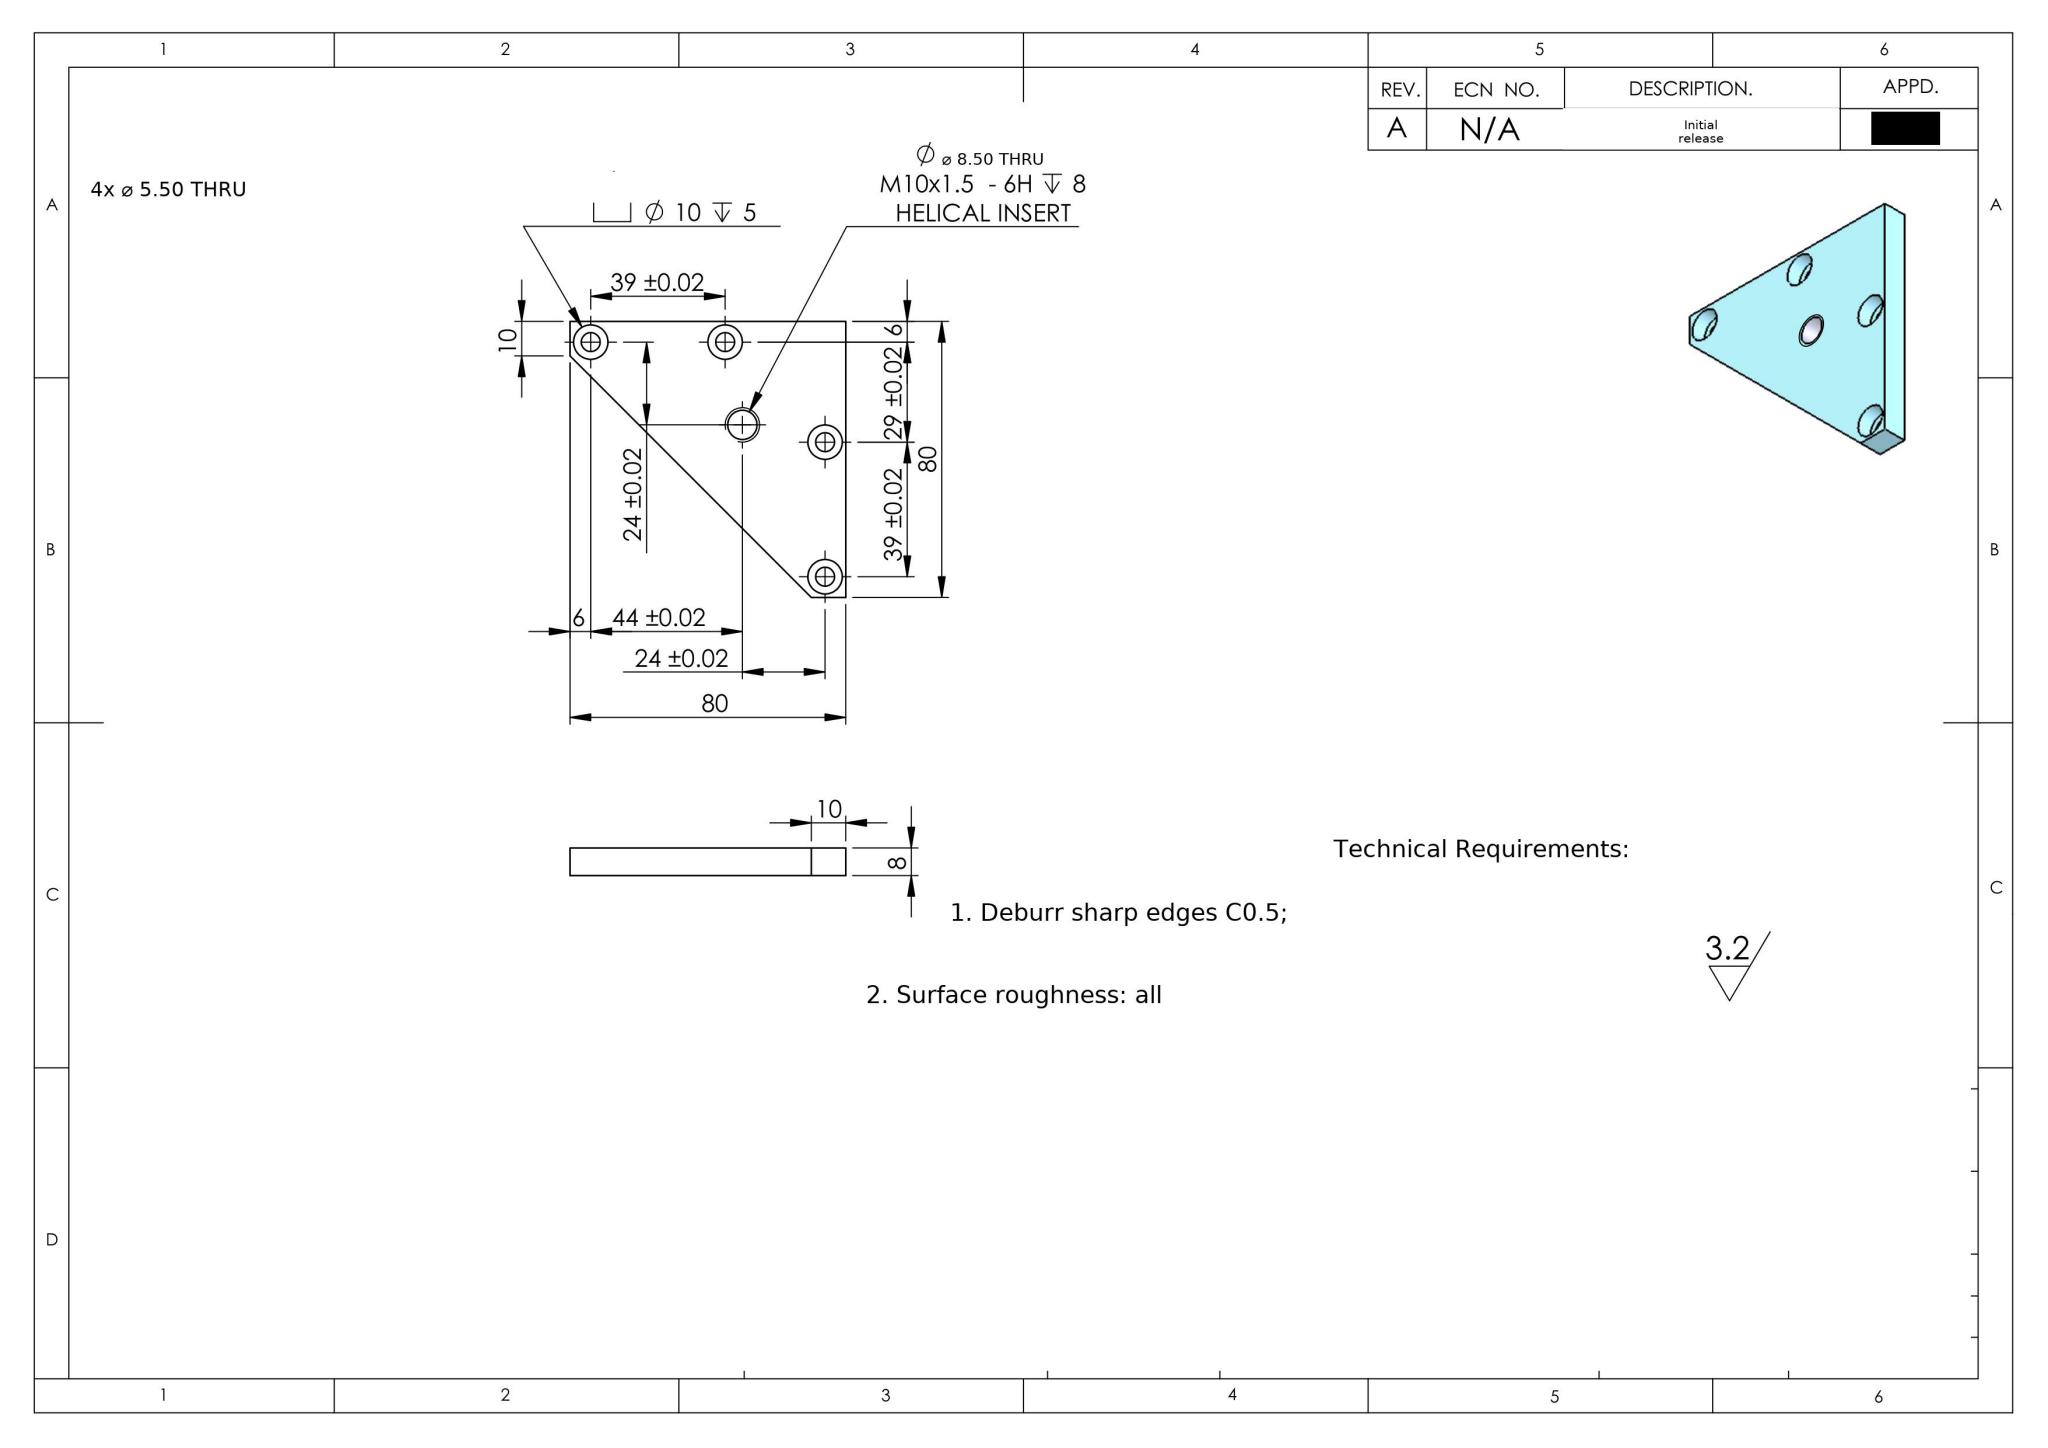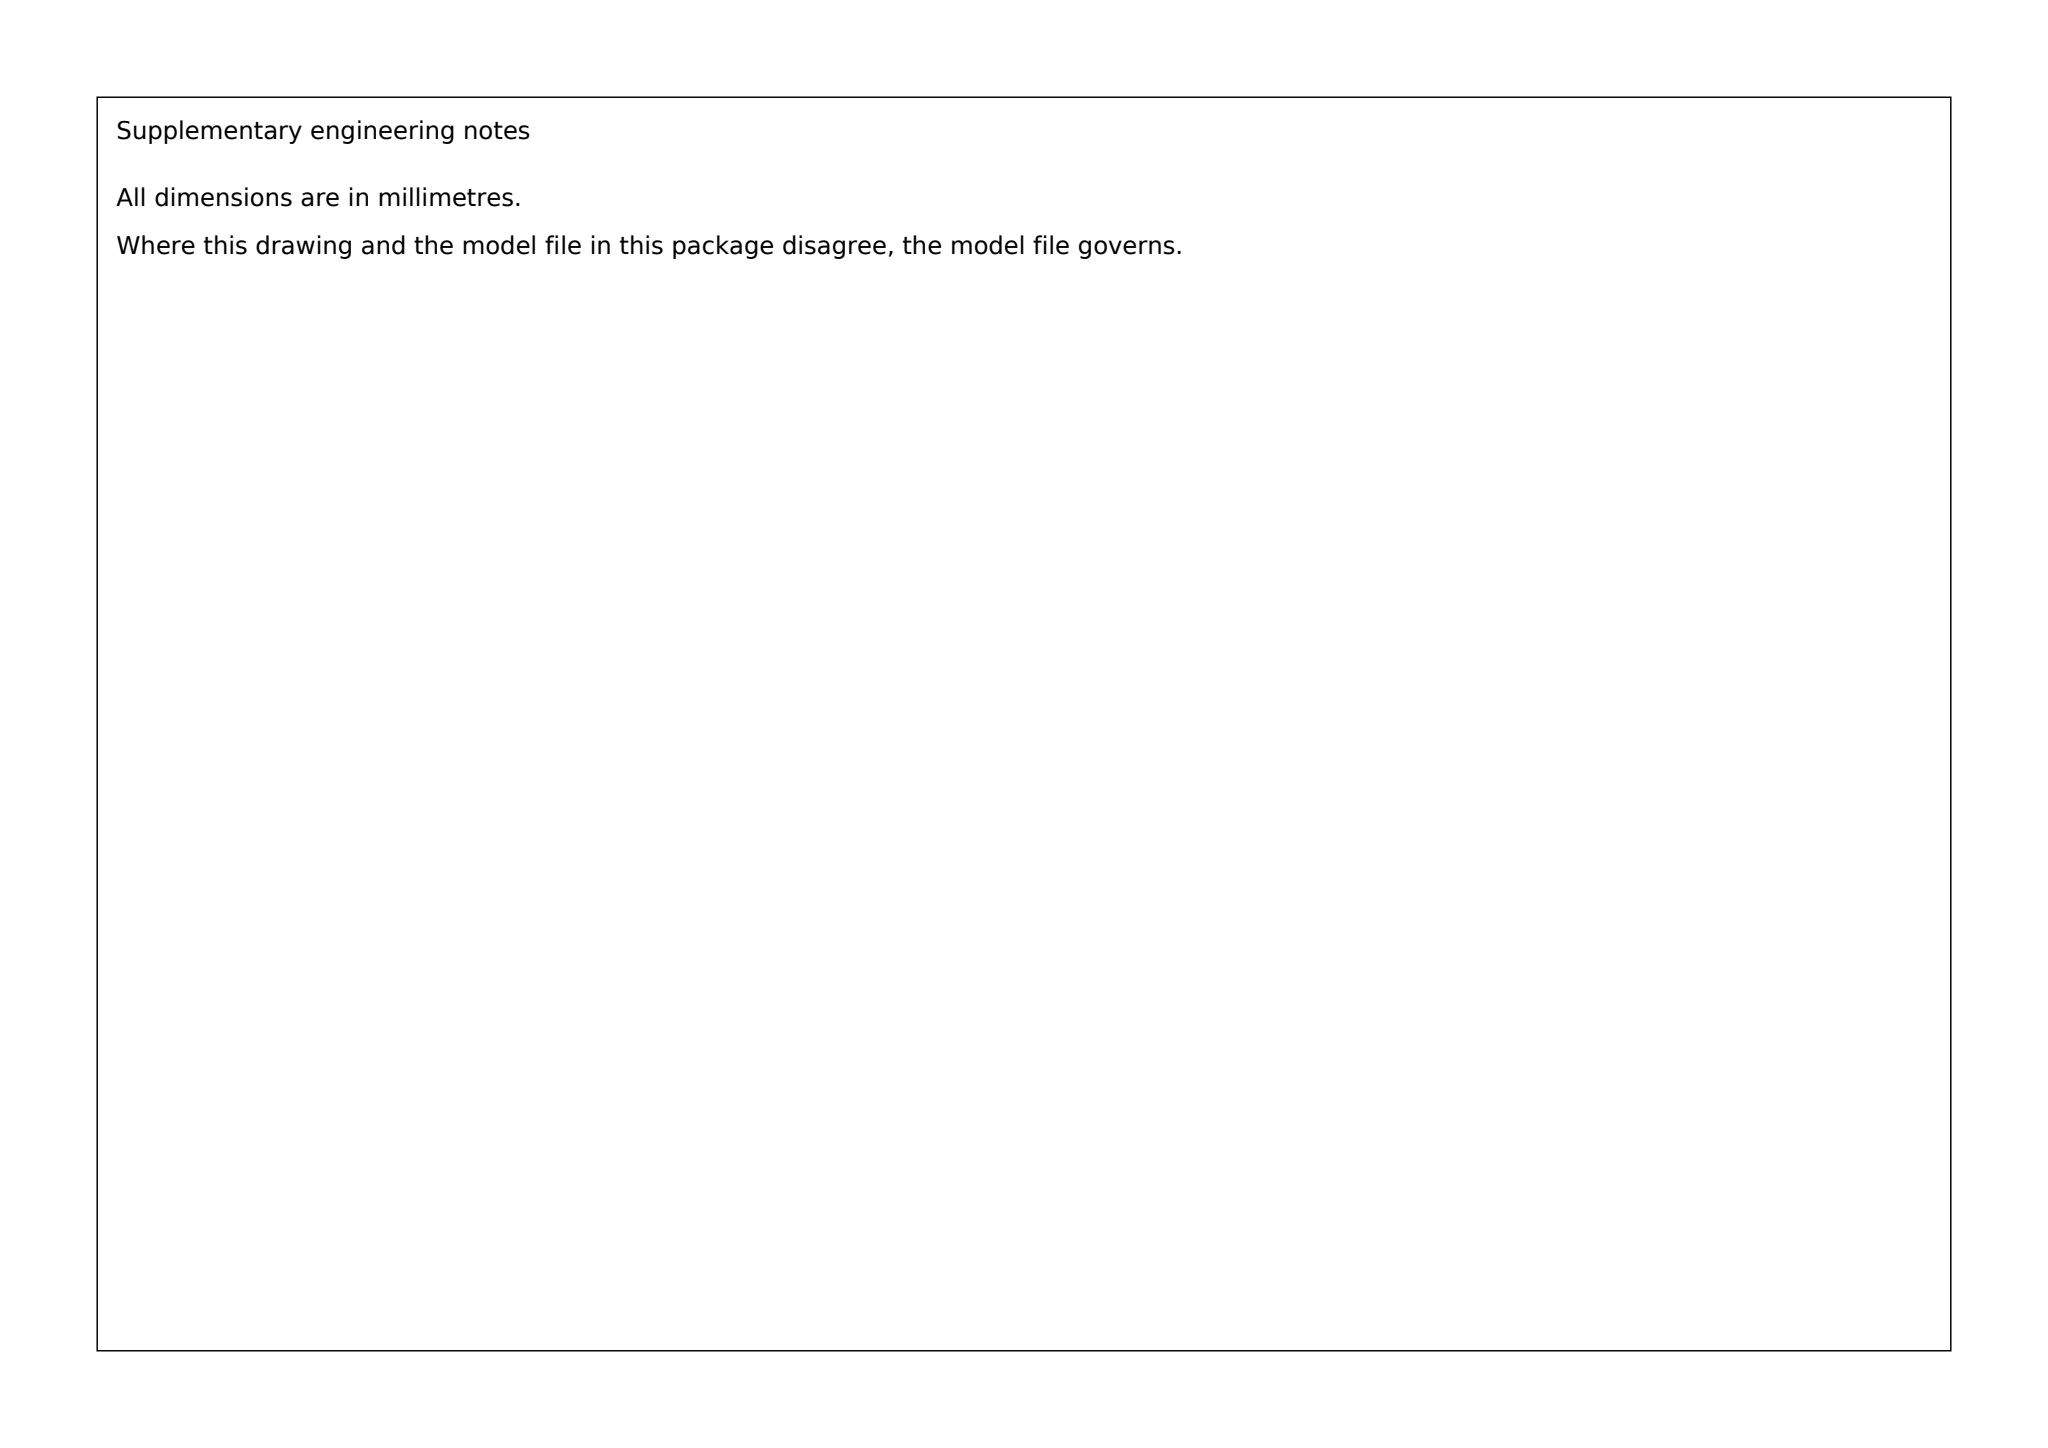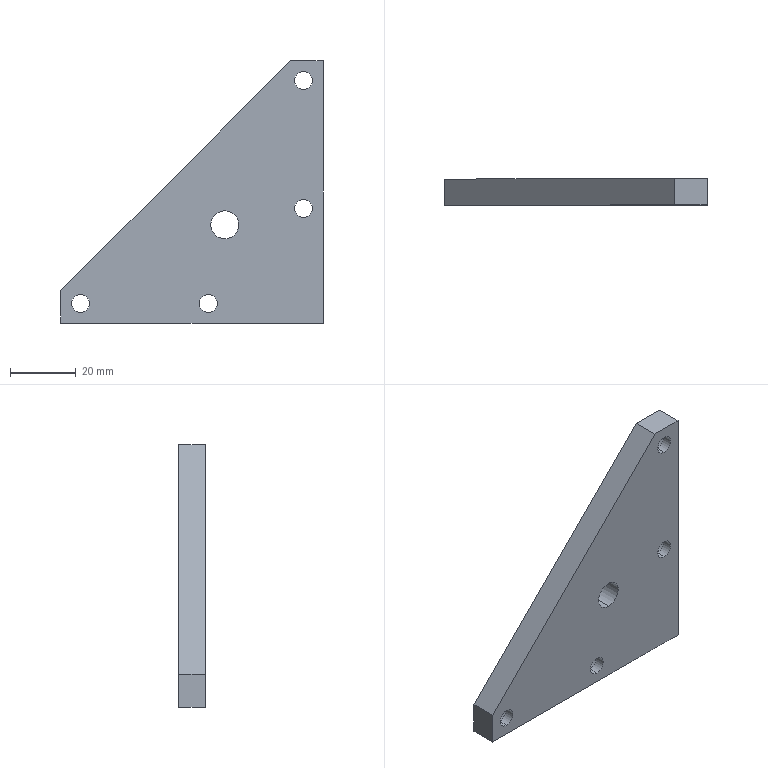Part | SolidWorks | mm | 1 solid | 29 faces | box 80 x 8 x 80 mm | volume 29290 mm3 | cylinder 18 | plane 11 | commonest cylinder face diameters 5.5 x8 10 x8 8.5 x2
build123d program:
from build123d import *

# Parameters (mm, degrees)
SKETCH1_W                                            = 80
SKETCH1_H                                            = 80
EXTRUDE1_DEPTH                                       = 8
COUNTERBORE_FOR_M5_HEX_SOCKET_HEAD_CAP_S_D           = 5.5
COUNTERBORE_FOR_M5_HEX_SOCKET_HEAD_CAP_S_CBORE_D     = 10
COUNTERBORE_FOR_M5_HEX_SOCKET_HEAD_CAP_S_CBORE_DEPTH = 5
M10_TAPPED_HOLE1_D                                   = 8.5
CUT_EXTRUDE1_REACH                                   = 115.42


with BuildPart() as part:
    # Sketch1 → Extrude1 (new body)
    with BuildSketch(Plane(origin=(0, 0, 0), x_dir=(1, 0, 0), z_dir=(0, 1, 0))):
        with Locations((40, 40)):
            Rectangle(SKETCH1_W, SKETCH1_H)
    extrude(amount=EXTRUDE1_DEPTH)

    # Counterbore for M5 Hex Socket Head Cap S (through all)
    with Locations(Plane(origin=(0, 8, 0), x_dir=(-1, 0, 0), z_dir=(0, 1, 0))):
        with Locations((-74, -45), (-74, -6), (-6, -6), (-6, -74), (-45, -74)):
            CounterBoreHole(COUNTERBORE_FOR_M5_HEX_SOCKET_HEAD_CAP_S_D / 2, COUNTERBORE_FOR_M5_HEX_SOCKET_HEAD_CAP_S_CBORE_D / 2, COUNTERBORE_FOR_M5_HEX_SOCKET_HEAD_CAP_S_CBORE_DEPTH)

    # M10 Tapped Hole1 (through all)
    with Locations(Plane(origin=(0, 8, 0), x_dir=(-1, 0, 0), z_dir=(0, 1, 0))):
        with Locations((-50, -50)):
            Hole(M10_TAPPED_HOLE1_D / 2)

    # Sketch8 → Cut-Extrude1 (cut, up to next)
    with BuildSketch(Plane(origin=(0, 8, 0), x_dir=(-1, 0, 0), z_dir=(0, 1, 0)), mode=Mode.PRIVATE) as cut_extrude1_sk1:
        Polygon((0, 0), (0, -70), (-70, 0), align=None)
    cut_extrude1_tool1 = extrude(cut_extrude1_sk1.sketch, amount=-CUT_EXTRUDE1_REACH, mode=Mode.PRIVATE) & part.part
    add(cut_extrude1_tool1.solids().sort_by_distance((23.333, 8, -23.333))[0], mode=Mode.SUBTRACT)


solid = part.part
STEP:
#1=CARTESIAN_POINT('',(50.,0.,-45.75));
#2=VERTEX_POINT('',#1);
#3=CARTESIAN_POINT('',(50.,0.,-54.25));
#4=VERTEX_POINT('',#3);
#5=CARTESIAN_POINT('',(50.,0.,-50.));
#6=DIRECTION('',(0.,-1.,0.));
#7=DIRECTION('',(0.,0.,-1.));
#8=AXIS2_PLACEMENT_3D('',#5,#6,#7);
#9=CIRCLE('',#8,4.25);
#10=EDGE_CURVE('',#2,#4,#9,.T.);
#11=ORIENTED_EDGE('',*,*,#10,.T.);
#12=CARTESIAN_POINT('',(50.,8.,-54.25));
#13=VERTEX_POINT('',#12);
#14=CARTESIAN_POINT('',(50.,8.,-54.25));
#15=DIRECTION('',(0.,1.,0.));
#16=VECTOR('',#15,1000.);
#17=LINE('',#14,#16);
#18=EDGE_CURVE('',#4,#13,#17,.T.);
#19=ORIENTED_EDGE('',*,*,#18,.T.);
#20=CARTESIAN_POINT('',(50.,8.,-45.75));
#21=VERTEX_POINT('',#20);
#22=CARTESIAN_POINT('',(50.,8.,-50.));
#23=DIRECTION('',(0.,1.,0.));
#24=DIRECTION('',(0.,0.,1.));
#25=AXIS2_PLACEMENT_3D('',#22,#23,#24);
#26=CIRCLE('',#25,4.25);
#27=EDGE_CURVE('',#13,#21,#26,.T.);
#28=ORIENTED_EDGE('',*,*,#27,.T.);
#29=CARTESIAN_POINT('',(50.,8.,-45.75));
#30=DIRECTION('',(0.,1.,0.));
#31=VECTOR('',#30,1000.);
#32=LINE('',#29,#31);
#33=EDGE_CURVE('',#2,#21,#32,.T.);
#34=ORIENTED_EDGE('',*,*,#33,.F.);
#35=EDGE_LOOP('',(#11,#19,#28,#34));
#36=FACE_OUTER_BOUND('',#35,.T.);
#37=CARTESIAN_POINT('',(50.,8.,-50.));
#38=DIRECTION('',(0.,1.,0.));
#39=DIRECTION('',(0.,0.,1.));
#40=AXIS2_PLACEMENT_3D('',#37,#38,#39);
#41=CYLINDRICAL_SURFACE('',#40,4.25);
#42=ADVANCED_FACE('',(#36),#41,.F.);
#43=CARTESIAN_POINT('',(74.,0.,-47.75));
#44=VERTEX_POINT('',#43);
#45=CARTESIAN_POINT('',(74.,0.,-42.25));
#46=VERTEX_POINT('',#45);
#47=CARTESIAN_POINT('',(74.,0.,-45.));
#48=DIRECTION('',(0.,1.,0.));
#49=DIRECTION('',(0.,0.,1.));
#50=AXIS2_PLACEMENT_3D('',#47,#48,#49);
#51=CIRCLE('',#50,2.75);
#52=EDGE_CURVE('',#44,#46,#51,.T.);
#53=ORIENTED_EDGE('',*,*,#52,.F.);
#54=CARTESIAN_POINT('',(74.,3.,-47.75));
#55=VERTEX_POINT('',#54);
#56=CARTESIAN_POINT('',(74.,8.,-47.75));
#57=DIRECTION('',(0.,1.,0.));
#58=VECTOR('',#57,1000.);
#59=LINE('',#56,#58);
#60=EDGE_CURVE('',#44,#55,#59,.T.);
#61=ORIENTED_EDGE('',*,*,#60,.T.);
#62=CARTESIAN_POINT('',(74.,3.,-42.25));
#63=VERTEX_POINT('',#62);
#64=CARTESIAN_POINT('',(74.,3.,-45.));
#65=DIRECTION('',(0.,1.,0.));
#66=DIRECTION('',(0.,0.,1.));
#67=AXIS2_PLACEMENT_3D('',#64,#65,#66);
#68=CIRCLE('',#67,2.75);
#69=EDGE_CURVE('',#55,#63,#68,.T.);
#70=ORIENTED_EDGE('',*,*,#69,.T.);
#71=CARTESIAN_POINT('',(74.,8.,-42.25));
#72=DIRECTION('',(0.,1.,0.));
#73=VECTOR('',#72,1000.);
#74=LINE('',#71,#73);
#75=EDGE_CURVE('',#46,#63,#74,.T.);
#76=ORIENTED_EDGE('',*,*,#75,.F.);
#77=EDGE_LOOP('',(#53,#61,#70,#76));
#78=FACE_OUTER_BOUND('',#77,.T.);
#79=CARTESIAN_POINT('',(74.,8.,-45.));
#80=DIRECTION('',(0.,1.,0.));
#81=DIRECTION('',(0.,0.,1.));
#82=AXIS2_PLACEMENT_3D('',#79,#80,#81);
#83=CYLINDRICAL_SURFACE('',#82,2.75);
#84=ADVANCED_FACE('',(#78),#83,.F.);
#85=CARTESIAN_POINT('',(74.,3.,-50.));
#86=VERTEX_POINT('',#85);
#87=CARTESIAN_POINT('',(74.,3.,-40.));
#88=VERTEX_POINT('',#87);
#89=CARTESIAN_POINT('',(74.,3.,-45.));
#90=DIRECTION('',(0.,1.,0.));
#91=DIRECTION('',(0.,0.,1.));
#92=AXIS2_PLACEMENT_3D('',#89,#90,#91);
#93=CIRCLE('',#92,5.);
#94=EDGE_CURVE('',#86,#88,#93,.T.);
#95=ORIENTED_EDGE('',*,*,#94,.F.);
#96=CARTESIAN_POINT('',(74.,8.,-50.));
#97=VERTEX_POINT('',#96);
#98=CARTESIAN_POINT('',(74.,8.,-50.));
#99=DIRECTION('',(0.,1.,0.));
#100=VECTOR('',#99,1000.);
#101=LINE('',#98,#100);
#102=EDGE_CURVE('',#86,#97,#101,.T.);
#103=ORIENTED_EDGE('',*,*,#102,.T.);
#104=CARTESIAN_POINT('',(74.,8.,-40.));
#105=VERTEX_POINT('',#104);
#106=CARTESIAN_POINT('',(74.,8.,-45.));
#107=DIRECTION('',(0.,1.,0.));
#108=DIRECTION('',(0.,0.,1.));
#109=AXIS2_PLACEMENT_3D('',#106,#107,#108);
#110=CIRCLE('',#109,5.);
#111=EDGE_CURVE('',#97,#105,#110,.T.);
#112=ORIENTED_EDGE('',*,*,#111,.T.);
#113=CARTESIAN_POINT('',(74.,8.,-40.));
#114=DIRECTION('',(0.,1.,0.));
#115=VECTOR('',#114,1000.);
#116=LINE('',#113,#115);
#117=EDGE_CURVE('',#88,#105,#116,.T.);
#118=ORIENTED_EDGE('',*,*,#117,.F.);
#119=EDGE_LOOP('',(#95,#103,#112,#118));
#120=FACE_OUTER_BOUND('',#119,.T.);
#121=CARTESIAN_POINT('',(74.,8.,-45.));
#122=DIRECTION('',(0.,1.,0.));
#123=DIRECTION('',(0.,0.,1.));
#124=AXIS2_PLACEMENT_3D('',#121,#122,#123);
#125=CYLINDRICAL_SURFACE('',#124,5.);
#126=ADVANCED_FACE('',(#120),#125,.F.);
#127=CARTESIAN_POINT('',(74.,0.,-8.75));
#128=VERTEX_POINT('',#127);
#129=CARTESIAN_POINT('',(74.,0.,-3.25));
#130=VERTEX_POINT('',#129);
#131=CARTESIAN_POINT('',(74.,0.,-6.));
#132=DIRECTION('',(0.,1.,0.));
#133=DIRECTION('',(0.,0.,1.));
#134=AXIS2_PLACEMENT_3D('',#131,#132,#133);
#135=CIRCLE('',#134,2.75);
#136=EDGE_CURVE('',#128,#130,#135,.T.);
#137=ORIENTED_EDGE('',*,*,#136,.F.);
#138=CARTESIAN_POINT('',(74.,3.,-8.75));
#139=VERTEX_POINT('',#138);
#140=CARTESIAN_POINT('',(74.,8.,-8.75));
#141=DIRECTION('',(0.,1.,0.));
#142=VECTOR('',#141,1000.);
#143=LINE('',#140,#142);
#144=EDGE_CURVE('',#128,#139,#143,.T.);
#145=ORIENTED_EDGE('',*,*,#144,.T.);
#146=CARTESIAN_POINT('',(74.,3.,-3.25));
#147=VERTEX_POINT('',#146);
#148=CARTESIAN_POINT('',(74.,3.,-6.));
#149=DIRECTION('',(0.,1.,0.));
#150=DIRECTION('',(0.,0.,1.));
#151=AXIS2_PLACEMENT_3D('',#148,#149,#150);
#152=CIRCLE('',#151,2.75);
#153=EDGE_CURVE('',#139,#147,#152,.T.);
#154=ORIENTED_EDGE('',*,*,#153,.T.);
#155=CARTESIAN_POINT('',(74.,8.,-3.25));
#156=DIRECTION('',(0.,1.,0.));
#157=VECTOR('',#156,1000.);
#158=LINE('',#155,#157);
#159=EDGE_CURVE('',#130,#147,#158,.T.);
#160=ORIENTED_EDGE('',*,*,#159,.F.);
#161=EDGE_LOOP('',(#137,#145,#154,#160));
#162=FACE_OUTER_BOUND('',#161,.T.);
#163=CARTESIAN_POINT('',(74.,8.,-6.));
#164=DIRECTION('',(0.,1.,0.));
#165=DIRECTION('',(0.,0.,1.));
#166=AXIS2_PLACEMENT_3D('',#163,#164,#165);
#167=CYLINDRICAL_SURFACE('',#166,2.75);
#168=ADVANCED_FACE('',(#162),#167,.F.);
#169=CARTESIAN_POINT('',(74.,3.,-11.));
#170=VERTEX_POINT('',#169);
#171=CARTESIAN_POINT('',(74.,3.,-1.));
#172=VERTEX_POINT('',#171);
#173=CARTESIAN_POINT('',(74.,3.,-6.));
#174=DIRECTION('',(0.,1.,0.));
#175=DIRECTION('',(0.,0.,1.));
#176=AXIS2_PLACEMENT_3D('',#173,#174,#175);
#177=CIRCLE('',#176,5.);
#178=EDGE_CURVE('',#170,#172,#177,.T.);
#179=ORIENTED_EDGE('',*,*,#178,.F.);
#180=CARTESIAN_POINT('',(74.,8.,-11.));
#181=VERTEX_POINT('',#180);
#182=CARTESIAN_POINT('',(74.,8.,-11.));
#183=DIRECTION('',(0.,1.,0.));
#184=VECTOR('',#183,1000.);
#185=LINE('',#182,#184);
#186=EDGE_CURVE('',#170,#181,#185,.T.);
#187=ORIENTED_EDGE('',*,*,#186,.T.);
#188=CARTESIAN_POINT('',(74.,8.,-1.));
#189=VERTEX_POINT('',#188);
#190=CARTESIAN_POINT('',(74.,8.,-6.));
#191=DIRECTION('',(0.,1.,0.));
#192=DIRECTION('',(0.,0.,1.));
#193=AXIS2_PLACEMENT_3D('',#190,#191,#192);
#194=CIRCLE('',#193,5.);
#195=EDGE_CURVE('',#181,#189,#194,.T.);
#196=ORIENTED_EDGE('',*,*,#195,.T.);
#197=CARTESIAN_POINT('',(74.,8.,-1.));
#198=DIRECTION('',(0.,1.,0.));
#199=VECTOR('',#198,1000.);
#200=LINE('',#197,#199);
#201=EDGE_CURVE('',#172,#189,#200,.T.);
#202=ORIENTED_EDGE('',*,*,#201,.F.);
#203=EDGE_LOOP('',(#179,#187,#196,#202));
#204=FACE_OUTER_BOUND('',#203,.T.);
#205=CARTESIAN_POINT('',(74.,8.,-6.));
#206=DIRECTION('',(0.,1.,0.));
#207=DIRECTION('',(0.,0.,1.));
#208=AXIS2_PLACEMENT_3D('',#205,#206,#207);
#209=CYLINDRICAL_SURFACE('',#208,5.);
#210=ADVANCED_FACE('',(#204),#209,.F.);
#211=CARTESIAN_POINT('',(6.,0.,-76.75));
#212=VERTEX_POINT('',#211);
#213=CARTESIAN_POINT('',(6.,0.,-71.25));
#214=VERTEX_POINT('',#213);
#215=CARTESIAN_POINT('',(6.,0.,-74.));
#216=DIRECTION('',(0.,1.,0.));
#217=DIRECTION('',(0.,0.,1.));
#218=AXIS2_PLACEMENT_3D('',#215,#216,#217);
#219=CIRCLE('',#218,2.75);
#220=EDGE_CURVE('',#212,#214,#219,.T.);
#221=ORIENTED_EDGE('',*,*,#220,.F.);
#222=CARTESIAN_POINT('',(6.,3.,-76.75));
#223=VERTEX_POINT('',#222);
#224=CARTESIAN_POINT('',(6.,8.,-76.75));
#225=DIRECTION('',(0.,1.,0.));
#226=VECTOR('',#225,1000.);
#227=LINE('',#224,#226);
#228=EDGE_CURVE('',#212,#223,#227,.T.);
#229=ORIENTED_EDGE('',*,*,#228,.T.);
#230=CARTESIAN_POINT('',(6.,3.,-71.25));
#231=VERTEX_POINT('',#230);
#232=CARTESIAN_POINT('',(6.,3.,-74.));
#233=DIRECTION('',(0.,1.,0.));
#234=DIRECTION('',(0.,0.,1.));
#235=AXIS2_PLACEMENT_3D('',#232,#233,#234);
#236=CIRCLE('',#235,2.75);
#237=EDGE_CURVE('',#223,#231,#236,.T.);
#238=ORIENTED_EDGE('',*,*,#237,.T.);
#239=CARTESIAN_POINT('',(6.,8.,-71.25));
#240=DIRECTION('',(0.,1.,0.));
#241=VECTOR('',#240,1000.);
#242=LINE('',#239,#241);
#243=EDGE_CURVE('',#214,#231,#242,.T.);
#244=ORIENTED_EDGE('',*,*,#243,.F.);
#245=EDGE_LOOP('',(#221,#229,#238,#244));
#246=FACE_OUTER_BOUND('',#245,.T.);
#247=CARTESIAN_POINT('',(6.,8.,-74.));
#248=DIRECTION('',(0.,1.,0.));
#249=DIRECTION('',(0.,0.,1.));
#250=AXIS2_PLACEMENT_3D('',#247,#248,#249);
#251=CYLINDRICAL_SURFACE('',#250,2.75);
#252=ADVANCED_FACE('',(#246),#251,.F.);
#253=CARTESIAN_POINT('',(6.,3.,-79.));
#254=VERTEX_POINT('',#253);
#255=CARTESIAN_POINT('',(6.,3.,-69.));
#256=VERTEX_POINT('',#255);
#257=CARTESIAN_POINT('',(6.,3.,-74.));
#258=DIRECTION('',(0.,1.,0.));
#259=DIRECTION('',(0.,0.,1.));
#260=AXIS2_PLACEMENT_3D('',#257,#258,#259);
#261=CIRCLE('',#260,5.);
#262=EDGE_CURVE('',#254,#256,#261,.T.);
#263=ORIENTED_EDGE('',*,*,#262,.F.);
#264=CARTESIAN_POINT('',(6.,8.,-79.));
#265=VERTEX_POINT('',#264);
#266=CARTESIAN_POINT('',(6.,8.,-79.));
#267=DIRECTION('',(0.,1.,0.));
#268=VECTOR('',#267,1000.);
#269=LINE('',#266,#268);
#270=EDGE_CURVE('',#254,#265,#269,.T.);
#271=ORIENTED_EDGE('',*,*,#270,.T.);
#272=CARTESIAN_POINT('',(6.,8.,-69.));
#273=VERTEX_POINT('',#272);
#274=CARTESIAN_POINT('',(6.,8.,-74.));
#275=DIRECTION('',(0.,1.,0.));
#276=DIRECTION('',(0.,0.,1.));
#277=AXIS2_PLACEMENT_3D('',#274,#275,#276);
#278=CIRCLE('',#277,5.);
#279=EDGE_CURVE('',#265,#273,#278,.T.);
#280=ORIENTED_EDGE('',*,*,#279,.T.);
#281=CARTESIAN_POINT('',(6.,8.,-69.));
#282=DIRECTION('',(0.,1.,0.));
#283=VECTOR('',#282,1000.);
#284=LINE('',#281,#283);
#285=EDGE_CURVE('',#256,#273,#284,.T.);
#286=ORIENTED_EDGE('',*,*,#285,.F.);
#287=EDGE_LOOP('',(#263,#271,#280,#286));
#288=FACE_OUTER_BOUND('',#287,.T.);
#289=CARTESIAN_POINT('',(6.,8.,-74.));
#290=DIRECTION('',(0.,1.,0.));
#291=DIRECTION('',(0.,0.,1.));
#292=AXIS2_PLACEMENT_3D('',#289,#290,#291);
#293=CYLINDRICAL_SURFACE('',#292,5.);
#294=ADVANCED_FACE('',(#288),#293,.F.);
#295=CARTESIAN_POINT('',(45.,0.,-76.75));
#296=VERTEX_POINT('',#295);
#297=CARTESIAN_POINT('',(45.,0.,-71.25));
#298=VERTEX_POINT('',#297);
#299=CARTESIAN_POINT('',(45.,0.,-74.));
#300=DIRECTION('',(0.,1.,0.));
#301=DIRECTION('',(0.,0.,1.));
#302=AXIS2_PLACEMENT_3D('',#299,#300,#301);
#303=CIRCLE('',#302,2.75);
#304=EDGE_CURVE('',#296,#298,#303,.T.);
#305=ORIENTED_EDGE('',*,*,#304,.F.);
#306=CARTESIAN_POINT('',(45.,3.,-76.75));
#307=VERTEX_POINT('',#306);
#308=CARTESIAN_POINT('',(45.,8.,-76.75));
#309=DIRECTION('',(0.,1.,0.));
#310=VECTOR('',#309,1000.);
#311=LINE('',#308,#310);
#312=EDGE_CURVE('',#296,#307,#311,.T.);
#313=ORIENTED_EDGE('',*,*,#312,.T.);
#314=CARTESIAN_POINT('',(45.,3.,-71.25));
#315=VERTEX_POINT('',#314);
#316=CARTESIAN_POINT('',(45.,3.,-74.));
#317=DIRECTION('',(0.,1.,0.));
#318=DIRECTION('',(0.,0.,1.));
#319=AXIS2_PLACEMENT_3D('',#316,#317,#318);
#320=CIRCLE('',#319,2.75);
#321=EDGE_CURVE('',#307,#315,#320,.T.);
#322=ORIENTED_EDGE('',*,*,#321,.T.);
#323=CARTESIAN_POINT('',(45.,8.,-71.25));
#324=DIRECTION('',(0.,1.,0.));
#325=VECTOR('',#324,1000.);
#326=LINE('',#323,#325);
#327=EDGE_CURVE('',#298,#315,#326,.T.);
#328=ORIENTED_EDGE('',*,*,#327,.F.);
#329=EDGE_LOOP('',(#305,#313,#322,#328));
#330=FACE_OUTER_BOUND('',#329,.T.);
#331=CARTESIAN_POINT('',(45.,8.,-74.));
#332=DIRECTION('',(0.,1.,0.));
#333=DIRECTION('',(0.,0.,1.));
#334=AXIS2_PLACEMENT_3D('',#331,#332,#333);
#335=CYLINDRICAL_SURFACE('',#334,2.75);
#336=ADVANCED_FACE('',(#330),#335,.F.);
#337=CARTESIAN_POINT('',(45.,3.,-79.));
#338=VERTEX_POINT('',#337);
#339=CARTESIAN_POINT('',(45.,3.,-69.));
#340=VERTEX_POINT('',#339);
#341=CARTESIAN_POINT('',(45.,3.,-74.));
#342=DIRECTION('',(0.,1.,0.));
#343=DIRECTION('',(0.,0.,1.));
#344=AXIS2_PLACEMENT_3D('',#341,#342,#343);
#345=CIRCLE('',#344,5.);
#346=EDGE_CURVE('',#338,#340,#345,.T.);
#347=ORIENTED_EDGE('',*,*,#346,.F.);
#348=CARTESIAN_POINT('',(45.,8.,-79.));
#349=VERTEX_POINT('',#348);
#350=CARTESIAN_POINT('',(45.,8.,-79.));
#351=DIRECTION('',(0.,1.,0.));
#352=VECTOR('',#351,1000.);
#353=LINE('',#350,#352);
#354=EDGE_CURVE('',#338,#349,#353,.T.);
#355=ORIENTED_EDGE('',*,*,#354,.T.);
#356=CARTESIAN_POINT('',(45.,8.,-69.));
#357=VERTEX_POINT('',#356);
#358=CARTESIAN_POINT('',(45.,8.,-74.));
#359=DIRECTION('',(0.,1.,0.));
#360=DIRECTION('',(0.,0.,1.));
#361=AXIS2_PLACEMENT_3D('',#358,#359,#360);
#362=CIRCLE('',#361,5.);
#363=EDGE_CURVE('',#349,#357,#362,.T.);
#364=ORIENTED_EDGE('',*,*,#363,.T.);
#365=CARTESIAN_POINT('',(45.,8.,-69.));
#366=DIRECTION('',(0.,1.,0.));
#367=VECTOR('',#366,1000.);
#368=LINE('',#365,#367);
#369=EDGE_CURVE('',#340,#357,#368,.T.);
#370=ORIENTED_EDGE('',*,*,#369,.F.);
#371=EDGE_LOOP('',(#347,#355,#364,#370));
#372=FACE_OUTER_BOUND('',#371,.T.);
#373=CARTESIAN_POINT('',(45.,8.,-74.));
#374=DIRECTION('',(0.,1.,0.));
#375=DIRECTION('',(0.,0.,1.));
#376=AXIS2_PLACEMENT_3D('',#373,#374,#375);
#377=CYLINDRICAL_SURFACE('',#376,5.);
#378=ADVANCED_FACE('',(#372),#377,.F.);
#379=CARTESIAN_POINT('',(0.,8.,-80.));
#380=VERTEX_POINT('',#379);
#381=CARTESIAN_POINT('',(0.,8.,-70.));
#382=VERTEX_POINT('',#381);
#383=CARTESIAN_POINT('',(0.,8.,0.));
#384=DIRECTION('',(0.,0.,1.));
#385=VECTOR('',#384,1000.);
#386=LINE('',#383,#385);
#387=EDGE_CURVE('',#380,#382,#386,.T.);
#388=ORIENTED_EDGE('',*,*,#387,.T.);
#389=CARTESIAN_POINT('',(70.,8.,0.));
#390=VERTEX_POINT('',#389);
#391=CARTESIAN_POINT('',(0.,8.,-70.));
#392=DIRECTION('',(-0.7071,0.,-0.7071));
#393=VECTOR('',#392,1000.);
#394=LINE('',#391,#393);
#395=EDGE_CURVE('',#390,#382,#394,.T.);
#396=ORIENTED_EDGE('',*,*,#395,.F.);
#397=CARTESIAN_POINT('',(80.,8.,0.));
#398=VERTEX_POINT('',#397);
#399=CARTESIAN_POINT('',(0.,8.,0.));
#400=DIRECTION('',(1.,0.,0.));
#401=VECTOR('',#400,1000.);
#402=LINE('',#399,#401);
#403=EDGE_CURVE('',#390,#398,#402,.T.);
#404=ORIENTED_EDGE('',*,*,#403,.T.);
#405=CARTESIAN_POINT('',(80.,8.,-80.));
#406=VERTEX_POINT('',#405);
#407=CARTESIAN_POINT('',(80.,8.,0.));
#408=DIRECTION('',(0.,0.,-1.));
#409=VECTOR('',#408,1000.);
#410=LINE('',#407,#409);
#411=EDGE_CURVE('',#398,#406,#410,.T.);
#412=ORIENTED_EDGE('',*,*,#411,.T.);
#413=CARTESIAN_POINT('',(0.,8.,-80.));
#414=DIRECTION('',(-1.,0.,0.));
#415=VECTOR('',#414,1000.);
#416=LINE('',#413,#415);
#417=EDGE_CURVE('',#406,#380,#416,.T.);
#418=ORIENTED_EDGE('',*,*,#417,.T.);
#419=EDGE_LOOP('',(#388,#396,#404,#412,#418));
#420=FACE_OUTER_BOUND('',#419,.T.);
#421=CARTESIAN_POINT('',(45.,8.,-74.));
#422=DIRECTION('',(0.,1.,0.));
#423=DIRECTION('',(0.,0.,1.));
#424=AXIS2_PLACEMENT_3D('',#421,#422,#423);
#425=CIRCLE('',#424,5.);
#426=EDGE_CURVE('',#357,#349,#425,.T.);
#427=ORIENTED_EDGE('',*,*,#426,.F.);
#428=ORIENTED_EDGE('',*,*,#363,.F.);
#429=EDGE_LOOP('',(#427,#428));
#430=FACE_BOUND('',#429,.T.);
#431=CARTESIAN_POINT('',(6.,8.,-74.));
#432=DIRECTION('',(0.,1.,0.));
#433=DIRECTION('',(0.,0.,1.));
#434=AXIS2_PLACEMENT_3D('',#431,#432,#433);
#435=CIRCLE('',#434,5.);
#436=EDGE_CURVE('',#273,#265,#435,.T.);
#437=ORIENTED_EDGE('',*,*,#436,.F.);
#438=ORIENTED_EDGE('',*,*,#279,.F.);
#439=EDGE_LOOP('',(#437,#438));
#440=FACE_BOUND('',#439,.T.);
#441=CARTESIAN_POINT('',(74.,8.,-6.));
#442=DIRECTION('',(0.,1.,0.));
#443=DIRECTION('',(0.,0.,1.));
#444=AXIS2_PLACEMENT_3D('',#441,#442,#443);
#445=CIRCLE('',#444,5.);
#446=EDGE_CURVE('',#189,#181,#445,.T.);
#447=ORIENTED_EDGE('',*,*,#446,.F.);
#448=ORIENTED_EDGE('',*,*,#195,.F.);
#449=EDGE_LOOP('',(#447,#448));
#450=FACE_BOUND('',#449,.T.);
#451=CARTESIAN_POINT('',(74.,8.,-45.));
#452=DIRECTION('',(0.,1.,0.));
#453=DIRECTION('',(0.,0.,1.));
#454=AXIS2_PLACEMENT_3D('',#451,#452,#453);
#455=CIRCLE('',#454,5.);
#456=EDGE_CURVE('',#105,#97,#455,.T.);
#457=ORIENTED_EDGE('',*,*,#456,.F.);
#458=ORIENTED_EDGE('',*,*,#111,.F.);
#459=EDGE_LOOP('',(#457,#458));
#460=FACE_BOUND('',#459,.T.);
#461=CARTESIAN_POINT('',(50.,8.,-50.));
#462=DIRECTION('',(0.,1.,0.));
#463=DIRECTION('',(0.,0.,1.));
#464=AXIS2_PLACEMENT_3D('',#461,#462,#463);
#465=CIRCLE('',#464,4.25);
#466=EDGE_CURVE('',#21,#13,#465,.T.);
#467=ORIENTED_EDGE('',*,*,#466,.F.);
#468=ORIENTED_EDGE('',*,*,#27,.F.);
#469=EDGE_LOOP('',(#467,#468));
#470=FACE_BOUND('',#469,.T.);
#471=CARTESIAN_POINT('',(0.,8.,-80.));
#472=DIRECTION('',(0.,-1.,0.));
#473=DIRECTION('',(0.,0.,-1.));
#474=AXIS2_PLACEMENT_3D('',#471,#472,#473);
#475=PLANE('',#474);
#476=ADVANCED_FACE('',(#420,#430,#440,#450,#460,#470),#475,.F.);
#477=CARTESIAN_POINT('',(70.,0.,0.));
#478=VERTEX_POINT('',#477);
#479=CARTESIAN_POINT('',(0.,0.,-70.));
#480=VERTEX_POINT('',#479);
#481=CARTESIAN_POINT('',(0.,0.,-70.));
#482=DIRECTION('',(-0.7071,0.,-0.7071));
#483=VECTOR('',#482,1000.);
#484=LINE('',#481,#483);
#485=EDGE_CURVE('',#478,#480,#484,.T.);
#486=ORIENTED_EDGE('',*,*,#485,.T.);
#487=CARTESIAN_POINT('',(0.,0.,-80.));
#488=VERTEX_POINT('',#487);
#489=CARTESIAN_POINT('',(0.,0.,0.));
#490=DIRECTION('',(0.,0.,1.));
#491=VECTOR('',#490,1000.);
#492=LINE('',#489,#491);
#493=EDGE_CURVE('',#488,#480,#492,.T.);
#494=ORIENTED_EDGE('',*,*,#493,.F.);
#495=CARTESIAN_POINT('',(80.,0.,-80.));
#496=VERTEX_POINT('',#495);
#497=CARTESIAN_POINT('',(0.,0.,-80.));
#498=DIRECTION('',(-1.,0.,0.));
#499=VECTOR('',#498,1000.);
#500=LINE('',#497,#499);
#501=EDGE_CURVE('',#496,#488,#500,.T.);
#502=ORIENTED_EDGE('',*,*,#501,.F.);
#503=CARTESIAN_POINT('',(80.,0.,0.));
#504=VERTEX_POINT('',#503);
#505=CARTESIAN_POINT('',(80.,0.,0.));
#506=DIRECTION('',(0.,0.,-1.));
#507=VECTOR('',#506,1000.);
#508=LINE('',#505,#507);
#509=EDGE_CURVE('',#504,#496,#508,.T.);
#510=ORIENTED_EDGE('',*,*,#509,.F.);
#511=CARTESIAN_POINT('',(0.,0.,0.));
#512=DIRECTION('',(1.,0.,0.));
#513=VECTOR('',#512,1000.);
#514=LINE('',#511,#513);
#515=EDGE_CURVE('',#478,#504,#514,.T.);
#516=ORIENTED_EDGE('',*,*,#515,.F.);
#517=EDGE_LOOP('',(#486,#494,#502,#510,#516));
#518=FACE_OUTER_BOUND('',#517,.T.);
#519=ORIENTED_EDGE('',*,*,#10,.F.);
#520=CARTESIAN_POINT('',(50.,0.,-50.));
#521=DIRECTION('',(0.,-1.,0.));
#522=DIRECTION('',(0.,0.,-1.));
#523=AXIS2_PLACEMENT_3D('',#520,#521,#522);
#524=CIRCLE('',#523,4.25);
#525=EDGE_CURVE('',#4,#2,#524,.T.);
#526=ORIENTED_EDGE('',*,*,#525,.F.);
#527=EDGE_LOOP('',(#519,#526));
#528=FACE_BOUND('',#527,.T.);
#529=CARTESIAN_POINT('',(74.,0.,-6.));
#530=DIRECTION('',(0.,1.,0.));
#531=DIRECTION('',(0.,0.,1.));
#532=AXIS2_PLACEMENT_3D('',#529,#530,#531);
#533=CIRCLE('',#532,2.75);
#534=EDGE_CURVE('',#130,#128,#533,.T.);
#535=ORIENTED_EDGE('',*,*,#534,.T.);
#536=ORIENTED_EDGE('',*,*,#136,.T.);
#537=EDGE_LOOP('',(#535,#536));
#538=FACE_BOUND('',#537,.T.);
#539=CARTESIAN_POINT('',(6.,0.,-74.));
#540=DIRECTION('',(0.,1.,0.));
#541=DIRECTION('',(0.,0.,1.));
#542=AXIS2_PLACEMENT_3D('',#539,#540,#541);
#543=CIRCLE('',#542,2.75);
#544=EDGE_CURVE('',#214,#212,#543,.T.);
#545=ORIENTED_EDGE('',*,*,#544,.T.);
#546=ORIENTED_EDGE('',*,*,#220,.T.);
#547=EDGE_LOOP('',(#545,#546));
#548=FACE_BOUND('',#547,.T.);
#549=CARTESIAN_POINT('',(45.,0.,-74.));
#550=DIRECTION('',(0.,1.,0.));
#551=DIRECTION('',(0.,0.,1.));
#552=AXIS2_PLACEMENT_3D('',#549,#550,#551);
#553=CIRCLE('',#552,2.75);
#554=EDGE_CURVE('',#298,#296,#553,.T.);
#555=ORIENTED_EDGE('',*,*,#554,.T.);
#556=ORIENTED_EDGE('',*,*,#304,.T.);
#557=EDGE_LOOP('',(#555,#556));
#558=FACE_BOUND('',#557,.T.);
#559=CARTESIAN_POINT('',(74.,0.,-45.));
#560=DIRECTION('',(0.,1.,0.));
#561=DIRECTION('',(0.,0.,1.));
#562=AXIS2_PLACEMENT_3D('',#559,#560,#561);
#563=CIRCLE('',#562,2.75);
#564=EDGE_CURVE('',#46,#44,#563,.T.);
#565=ORIENTED_EDGE('',*,*,#564,.T.);
#566=ORIENTED_EDGE('',*,*,#52,.T.);
#567=EDGE_LOOP('',(#565,#566));
#568=FACE_BOUND('',#567,.T.);
#569=CARTESIAN_POINT('',(0.,0.,-80.));
#570=DIRECTION('',(0.,-1.,0.));
#571=DIRECTION('',(0.,0.,-1.));
#572=AXIS2_PLACEMENT_3D('',#569,#570,#571);
#573=PLANE('',#572);
#574=ADVANCED_FACE('',(#518,#528,#538,#548,#558,#568),#573,.T.);
#575=ORIENTED_EDGE('',*,*,#493,.T.);
#576=CARTESIAN_POINT('',(0.,-0.001,-70.));
#577=DIRECTION('',(0.,1.,0.));
#578=VECTOR('',#577,1000.);
#579=LINE('',#576,#578);
#580=EDGE_CURVE('',#480,#382,#579,.T.);
#581=ORIENTED_EDGE('',*,*,#580,.T.);
#582=ORIENTED_EDGE('',*,*,#387,.F.);
#583=CARTESIAN_POINT('',(0.,8.,-80.));
#584=DIRECTION('',(0.,-1.,0.));
#585=VECTOR('',#584,1000.);
#586=LINE('',#583,#585);
#587=EDGE_CURVE('',#380,#488,#586,.T.);
#588=ORIENTED_EDGE('',*,*,#587,.T.);
#589=EDGE_LOOP('',(#575,#581,#582,#588));
#590=FACE_OUTER_BOUND('',#589,.T.);
#591=CARTESIAN_POINT('',(0.,8.,0.));
#592=DIRECTION('',(1.,0.,0.));
#593=DIRECTION('',(0.,0.,-1.));
#594=AXIS2_PLACEMENT_3D('',#591,#592,#593);
#595=PLANE('',#594);
#596=ADVANCED_FACE('',(#590),#595,.F.);
#597=ORIENTED_EDGE('',*,*,#403,.F.);
#598=CARTESIAN_POINT('',(70.,-0.001,0.));
#599=DIRECTION('',(0.,1.,0.));
#600=VECTOR('',#599,1000.);
#601=LINE('',#598,#600);
#602=EDGE_CURVE('',#478,#390,#601,.T.);
#603=ORIENTED_EDGE('',*,*,#602,.F.);
#604=ORIENTED_EDGE('',*,*,#515,.T.);
#605=CARTESIAN_POINT('',(80.,8.,0.));
#606=DIRECTION('',(0.,-1.,0.));
#607=VECTOR('',#606,1000.);
#608=LINE('',#605,#607);
#609=EDGE_CURVE('',#398,#504,#608,.T.);
#610=ORIENTED_EDGE('',*,*,#609,.F.);
#611=EDGE_LOOP('',(#597,#603,#604,#610));
#612=FACE_OUTER_BOUND('',#611,.T.);
#613=CARTESIAN_POINT('',(0.,8.,0.));
#614=DIRECTION('',(0.,0.,-1.));
#615=DIRECTION('',(-1.,0.,0.));
#616=AXIS2_PLACEMENT_3D('',#613,#614,#615);
#617=PLANE('',#616);
#618=ADVANCED_FACE('',(#612),#617,.F.);
#619=ORIENTED_EDGE('',*,*,#509,.T.);
#620=CARTESIAN_POINT('',(80.,8.,-80.));
#621=DIRECTION('',(0.,-1.,0.));
#622=VECTOR('',#621,1000.);
#623=LINE('',#620,#622);
#624=EDGE_CURVE('',#406,#496,#623,.T.);
#625=ORIENTED_EDGE('',*,*,#624,.F.);
#626=ORIENTED_EDGE('',*,*,#411,.F.);
#627=ORIENTED_EDGE('',*,*,#609,.T.);
#628=EDGE_LOOP('',(#619,#625,#626,#627));
#629=FACE_OUTER_BOUND('',#628,.T.);
#630=CARTESIAN_POINT('',(80.,8.,0.));
#631=DIRECTION('',(-1.,0.,0.));
#632=DIRECTION('',(0.,0.,1.));
#633=AXIS2_PLACEMENT_3D('',#630,#631,#632);
#634=PLANE('',#633);
#635=ADVANCED_FACE('',(#629),#634,.F.);
#636=ORIENTED_EDGE('',*,*,#501,.T.);
#637=ORIENTED_EDGE('',*,*,#587,.F.);
#638=ORIENTED_EDGE('',*,*,#417,.F.);
#639=ORIENTED_EDGE('',*,*,#624,.T.);
#640=EDGE_LOOP('',(#636,#637,#638,#639));
#641=FACE_OUTER_BOUND('',#640,.T.);
#642=CARTESIAN_POINT('',(0.,8.,-80.));
#643=DIRECTION('',(0.,0.,1.));
#644=DIRECTION('',(1.,0.,0.));
#645=AXIS2_PLACEMENT_3D('',#642,#643,#644);
#646=PLANE('',#645);
#647=ADVANCED_FACE('',(#641),#646,.F.);
#648=ORIENTED_EDGE('',*,*,#354,.F.);
#649=CARTESIAN_POINT('',(45.,3.,-74.));
#650=DIRECTION('',(0.,1.,0.));
#651=DIRECTION('',(0.,0.,1.));
#652=AXIS2_PLACEMENT_3D('',#649,#650,#651);
#653=CIRCLE('',#652,5.);
#654=EDGE_CURVE('',#340,#338,#653,.T.);
#655=ORIENTED_EDGE('',*,*,#654,.F.);
#656=ORIENTED_EDGE('',*,*,#369,.T.);
#657=ORIENTED_EDGE('',*,*,#426,.T.);
#658=EDGE_LOOP('',(#648,#655,#656,#657));
#659=FACE_OUTER_BOUND('',#658,.T.);
#660=CARTESIAN_POINT('',(45.,8.,-74.));
#661=DIRECTION('',(0.,1.,0.));
#662=DIRECTION('',(0.,0.,1.));
#663=AXIS2_PLACEMENT_3D('',#660,#661,#662);
#664=CYLINDRICAL_SURFACE('',#663,5.);
#665=ADVANCED_FACE('',(#659),#664,.F.);
#666=CARTESIAN_POINT('',(45.,3.,-74.));
#667=DIRECTION('',(0.,1.,0.));
#668=DIRECTION('',(0.,0.,1.));
#669=AXIS2_PLACEMENT_3D('',#666,#667,#668);
#670=CIRCLE('',#669,2.75);
#671=EDGE_CURVE('',#315,#307,#670,.T.);
#672=ORIENTED_EDGE('',*,*,#671,.F.);
#673=ORIENTED_EDGE('',*,*,#321,.F.);
#674=EDGE_LOOP('',(#672,#673));
#675=FACE_BOUND('',#674,.T.);
#676=ORIENTED_EDGE('',*,*,#654,.T.);
#677=ORIENTED_EDGE('',*,*,#346,.T.);
#678=EDGE_LOOP('',(#676,#677));
#679=FACE_OUTER_BOUND('',#678,.T.);
#680=CARTESIAN_POINT('',(47.75,3.,-74.));
#681=DIRECTION('',(0.,-1.,0.));
#682=DIRECTION('',(0.,0.,-1.));
#683=AXIS2_PLACEMENT_3D('',#680,#681,#682);
#684=PLANE('',#683);
#685=ADVANCED_FACE('',(#675,#679),#684,.F.);
#686=ORIENTED_EDGE('',*,*,#312,.F.);
#687=ORIENTED_EDGE('',*,*,#554,.F.);
#688=ORIENTED_EDGE('',*,*,#327,.T.);
#689=ORIENTED_EDGE('',*,*,#671,.T.);
#690=EDGE_LOOP('',(#686,#687,#688,#689));
#691=FACE_OUTER_BOUND('',#690,.T.);
#692=CARTESIAN_POINT('',(45.,8.,-74.));
#693=DIRECTION('',(0.,1.,0.));
#694=DIRECTION('',(0.,0.,1.));
#695=AXIS2_PLACEMENT_3D('',#692,#693,#694);
#696=CYLINDRICAL_SURFACE('',#695,2.75);
#697=ADVANCED_FACE('',(#691),#696,.F.);
#698=ORIENTED_EDGE('',*,*,#270,.F.);
#699=CARTESIAN_POINT('',(6.,3.,-74.));
#700=DIRECTION('',(0.,1.,0.));
#701=DIRECTION('',(0.,0.,1.));
#702=AXIS2_PLACEMENT_3D('',#699,#700,#701);
#703=CIRCLE('',#702,5.);
#704=EDGE_CURVE('',#256,#254,#703,.T.);
#705=ORIENTED_EDGE('',*,*,#704,.F.);
#706=ORIENTED_EDGE('',*,*,#285,.T.);
#707=ORIENTED_EDGE('',*,*,#436,.T.);
#708=EDGE_LOOP('',(#698,#705,#706,#707));
#709=FACE_OUTER_BOUND('',#708,.T.);
#710=CARTESIAN_POINT('',(6.,8.,-74.));
#711=DIRECTION('',(0.,1.,0.));
#712=DIRECTION('',(0.,0.,1.));
#713=AXIS2_PLACEMENT_3D('',#710,#711,#712);
#714=CYLINDRICAL_SURFACE('',#713,5.);
#715=ADVANCED_FACE('',(#709),#714,.F.);
#716=CARTESIAN_POINT('',(6.,3.,-74.));
#717=DIRECTION('',(0.,1.,0.));
#718=DIRECTION('',(0.,0.,1.));
#719=AXIS2_PLACEMENT_3D('',#716,#717,#718);
#720=CIRCLE('',#719,2.75);
#721=EDGE_CURVE('',#231,#223,#720,.T.);
#722=ORIENTED_EDGE('',*,*,#721,.F.);
#723=ORIENTED_EDGE('',*,*,#237,.F.);
#724=EDGE_LOOP('',(#722,#723));
#725=FACE_BOUND('',#724,.T.);
#726=ORIENTED_EDGE('',*,*,#704,.T.);
#727=ORIENTED_EDGE('',*,*,#262,.T.);
#728=EDGE_LOOP('',(#726,#727));
#729=FACE_OUTER_BOUND('',#728,.T.);
#730=CARTESIAN_POINT('',(8.75,3.,-74.));
#731=DIRECTION('',(0.,-1.,0.));
#732=DIRECTION('',(0.,0.,-1.));
#733=AXIS2_PLACEMENT_3D('',#730,#731,#732);
#734=PLANE('',#733);
#735=ADVANCED_FACE('',(#725,#729),#734,.F.);
#736=ORIENTED_EDGE('',*,*,#228,.F.);
#737=ORIENTED_EDGE('',*,*,#544,.F.);
#738=ORIENTED_EDGE('',*,*,#243,.T.);
#739=ORIENTED_EDGE('',*,*,#721,.T.);
#740=EDGE_LOOP('',(#736,#737,#738,#739));
#741=FACE_OUTER_BOUND('',#740,.T.);
#742=CARTESIAN_POINT('',(6.,8.,-74.));
#743=DIRECTION('',(0.,1.,0.));
#744=DIRECTION('',(0.,0.,1.));
#745=AXIS2_PLACEMENT_3D('',#742,#743,#744);
#746=CYLINDRICAL_SURFACE('',#745,2.75);
#747=ADVANCED_FACE('',(#741),#746,.F.);
#748=ORIENTED_EDGE('',*,*,#186,.F.);
#749=CARTESIAN_POINT('',(74.,3.,-6.));
#750=DIRECTION('',(0.,1.,0.));
#751=DIRECTION('',(0.,0.,1.));
#752=AXIS2_PLACEMENT_3D('',#749,#750,#751);
#753=CIRCLE('',#752,5.);
#754=EDGE_CURVE('',#172,#170,#753,.T.);
#755=ORIENTED_EDGE('',*,*,#754,.F.);
#756=ORIENTED_EDGE('',*,*,#201,.T.);
#757=ORIENTED_EDGE('',*,*,#446,.T.);
#758=EDGE_LOOP('',(#748,#755,#756,#757));
#759=FACE_OUTER_BOUND('',#758,.T.);
#760=CARTESIAN_POINT('',(74.,8.,-6.));
#761=DIRECTION('',(0.,1.,0.));
#762=DIRECTION('',(0.,0.,1.));
#763=AXIS2_PLACEMENT_3D('',#760,#761,#762);
#764=CYLINDRICAL_SURFACE('',#763,5.);
#765=ADVANCED_FACE('',(#759),#764,.F.);
#766=CARTESIAN_POINT('',(74.,3.,-6.));
#767=DIRECTION('',(0.,1.,0.));
#768=DIRECTION('',(0.,0.,1.));
#769=AXIS2_PLACEMENT_3D('',#766,#767,#768);
#770=CIRCLE('',#769,2.75);
#771=EDGE_CURVE('',#147,#139,#770,.T.);
#772=ORIENTED_EDGE('',*,*,#771,.F.);
#773=ORIENTED_EDGE('',*,*,#153,.F.);
#774=EDGE_LOOP('',(#772,#773));
#775=FACE_BOUND('',#774,.T.);
#776=ORIENTED_EDGE('',*,*,#754,.T.);
#777=ORIENTED_EDGE('',*,*,#178,.T.);
#778=EDGE_LOOP('',(#776,#777));
#779=FACE_OUTER_BOUND('',#778,.T.);
#780=CARTESIAN_POINT('',(76.75,3.,-6.));
#781=DIRECTION('',(0.,-1.,0.));
#782=DIRECTION('',(0.,0.,-1.));
#783=AXIS2_PLACEMENT_3D('',#780,#781,#782);
#784=PLANE('',#783);
#785=ADVANCED_FACE('',(#775,#779),#784,.F.);
#786=ORIENTED_EDGE('',*,*,#144,.F.);
#787=ORIENTED_EDGE('',*,*,#534,.F.);
#788=ORIENTED_EDGE('',*,*,#159,.T.);
#789=ORIENTED_EDGE('',*,*,#771,.T.);
#790=EDGE_LOOP('',(#786,#787,#788,#789));
#791=FACE_OUTER_BOUND('',#790,.T.);
#792=CARTESIAN_POINT('',(74.,8.,-6.));
#793=DIRECTION('',(0.,1.,0.));
#794=DIRECTION('',(0.,0.,1.));
#795=AXIS2_PLACEMENT_3D('',#792,#793,#794);
#796=CYLINDRICAL_SURFACE('',#795,2.75);
#797=ADVANCED_FACE('',(#791),#796,.F.);
#798=ORIENTED_EDGE('',*,*,#102,.F.);
#799=CARTESIAN_POINT('',(74.,3.,-45.));
#800=DIRECTION('',(0.,1.,0.));
#801=DIRECTION('',(0.,0.,1.));
#802=AXIS2_PLACEMENT_3D('',#799,#800,#801);
#803=CIRCLE('',#802,5.);
#804=EDGE_CURVE('',#88,#86,#803,.T.);
#805=ORIENTED_EDGE('',*,*,#804,.F.);
#806=ORIENTED_EDGE('',*,*,#117,.T.);
#807=ORIENTED_EDGE('',*,*,#456,.T.);
#808=EDGE_LOOP('',(#798,#805,#806,#807));
#809=FACE_OUTER_BOUND('',#808,.T.);
#810=CARTESIAN_POINT('',(74.,8.,-45.));
#811=DIRECTION('',(0.,1.,0.));
#812=DIRECTION('',(0.,0.,1.));
#813=AXIS2_PLACEMENT_3D('',#810,#811,#812);
#814=CYLINDRICAL_SURFACE('',#813,5.);
#815=ADVANCED_FACE('',(#809),#814,.F.);
#816=CARTESIAN_POINT('',(74.,3.,-45.));
#817=DIRECTION('',(0.,1.,0.));
#818=DIRECTION('',(0.,0.,1.));
#819=AXIS2_PLACEMENT_3D('',#816,#817,#818);
#820=CIRCLE('',#819,2.75);
#821=EDGE_CURVE('',#63,#55,#820,.T.);
#822=ORIENTED_EDGE('',*,*,#821,.F.);
#823=ORIENTED_EDGE('',*,*,#69,.F.);
#824=EDGE_LOOP('',(#822,#823));
#825=FACE_BOUND('',#824,.T.);
#826=ORIENTED_EDGE('',*,*,#804,.T.);
#827=ORIENTED_EDGE('',*,*,#94,.T.);
#828=EDGE_LOOP('',(#826,#827));
#829=FACE_OUTER_BOUND('',#828,.T.);
#830=CARTESIAN_POINT('',(76.75,3.,-45.));
#831=DIRECTION('',(0.,-1.,0.));
#832=DIRECTION('',(0.,0.,-1.));
#833=AXIS2_PLACEMENT_3D('',#830,#831,#832);
#834=PLANE('',#833);
#835=ADVANCED_FACE('',(#825,#829),#834,.F.);
#836=ORIENTED_EDGE('',*,*,#60,.F.);
#837=ORIENTED_EDGE('',*,*,#564,.F.);
#838=ORIENTED_EDGE('',*,*,#75,.T.);
#839=ORIENTED_EDGE('',*,*,#821,.T.);
#840=EDGE_LOOP('',(#836,#837,#838,#839));
#841=FACE_OUTER_BOUND('',#840,.T.);
#842=CARTESIAN_POINT('',(74.,8.,-45.));
#843=DIRECTION('',(0.,1.,0.));
#844=DIRECTION('',(0.,0.,1.));
#845=AXIS2_PLACEMENT_3D('',#842,#843,#844);
#846=CYLINDRICAL_SURFACE('',#845,2.75);
#847=ADVANCED_FACE('',(#841),#846,.F.);
#848=ORIENTED_EDGE('',*,*,#18,.F.);
#849=ORIENTED_EDGE('',*,*,#525,.T.);
#850=ORIENTED_EDGE('',*,*,#33,.T.);
#851=ORIENTED_EDGE('',*,*,#466,.T.);
#852=EDGE_LOOP('',(#848,#849,#850,#851));
#853=FACE_OUTER_BOUND('',#852,.T.);
#854=CARTESIAN_POINT('',(50.,8.,-50.));
#855=DIRECTION('',(0.,1.,0.));
#856=DIRECTION('',(0.,0.,1.));
#857=AXIS2_PLACEMENT_3D('',#854,#855,#856);
#858=CYLINDRICAL_SURFACE('',#857,4.25);
#859=ADVANCED_FACE('',(#853),#858,.F.);
#860=ORIENTED_EDGE('',*,*,#602,.T.);
#861=ORIENTED_EDGE('',*,*,#395,.T.);
#862=ORIENTED_EDGE('',*,*,#580,.F.);
#863=ORIENTED_EDGE('',*,*,#485,.F.);
#864=EDGE_LOOP('',(#860,#861,#862,#863));
#865=FACE_OUTER_BOUND('',#864,.T.);
#866=CARTESIAN_POINT('',(0.,-0.001,-70.));
#867=DIRECTION('',(0.7071,0.,-0.7071));
#868=DIRECTION('',(-0.7071,0.,-0.7071));
#869=AXIS2_PLACEMENT_3D('',#866,#867,#868);
#870=PLANE('',#869);
#871=ADVANCED_FACE('',(#865),#870,.F.);
#872=CLOSED_SHELL('',(#42,#84,#126,#168,#210,#252,#294,#336,#378,#476,#574,#596,#618,#635,#647,#665,#685,#697,#715,#735,#747,#765,#785,#797,#815,#835,#847,#859,#871));
#873=MANIFOLD_SOLID_BREP('',#872);
#874=CARTESIAN_POINT('',(0.,0.,0.));
#875=DIRECTION('',(0.,0.,1.));
#876=DIRECTION('',(1.,0.,0.));
#877=AXIS2_PLACEMENT_3D('',#874,#875,#876);
#878=(LENGTH_UNIT()NAMED_UNIT(*)SI_UNIT(.MILLI.,.METRE.));
#879=UNCERTAINTY_MEASURE_WITH_UNIT(LENGTH_MEASURE(0.00001),#878,'','');
#880=(NAMED_UNIT(*)PLANE_ANGLE_UNIT()SI_UNIT($,.RADIAN.));
#881=(NAMED_UNIT(*)SI_UNIT($,.STERADIAN.)SOLID_ANGLE_UNIT());
#882=(GEOMETRIC_REPRESENTATION_CONTEXT(3)GLOBAL_UNCERTAINTY_ASSIGNED_CONTEXT((#879))GLOBAL_UNIT_ASSIGNED_CONTEXT((#878,#880,#881))REPRESENTATION_CONTEXT('',''));
#883=ADVANCED_BREP_SHAPE_REPRESENTATION('',(#873,#877),#882);